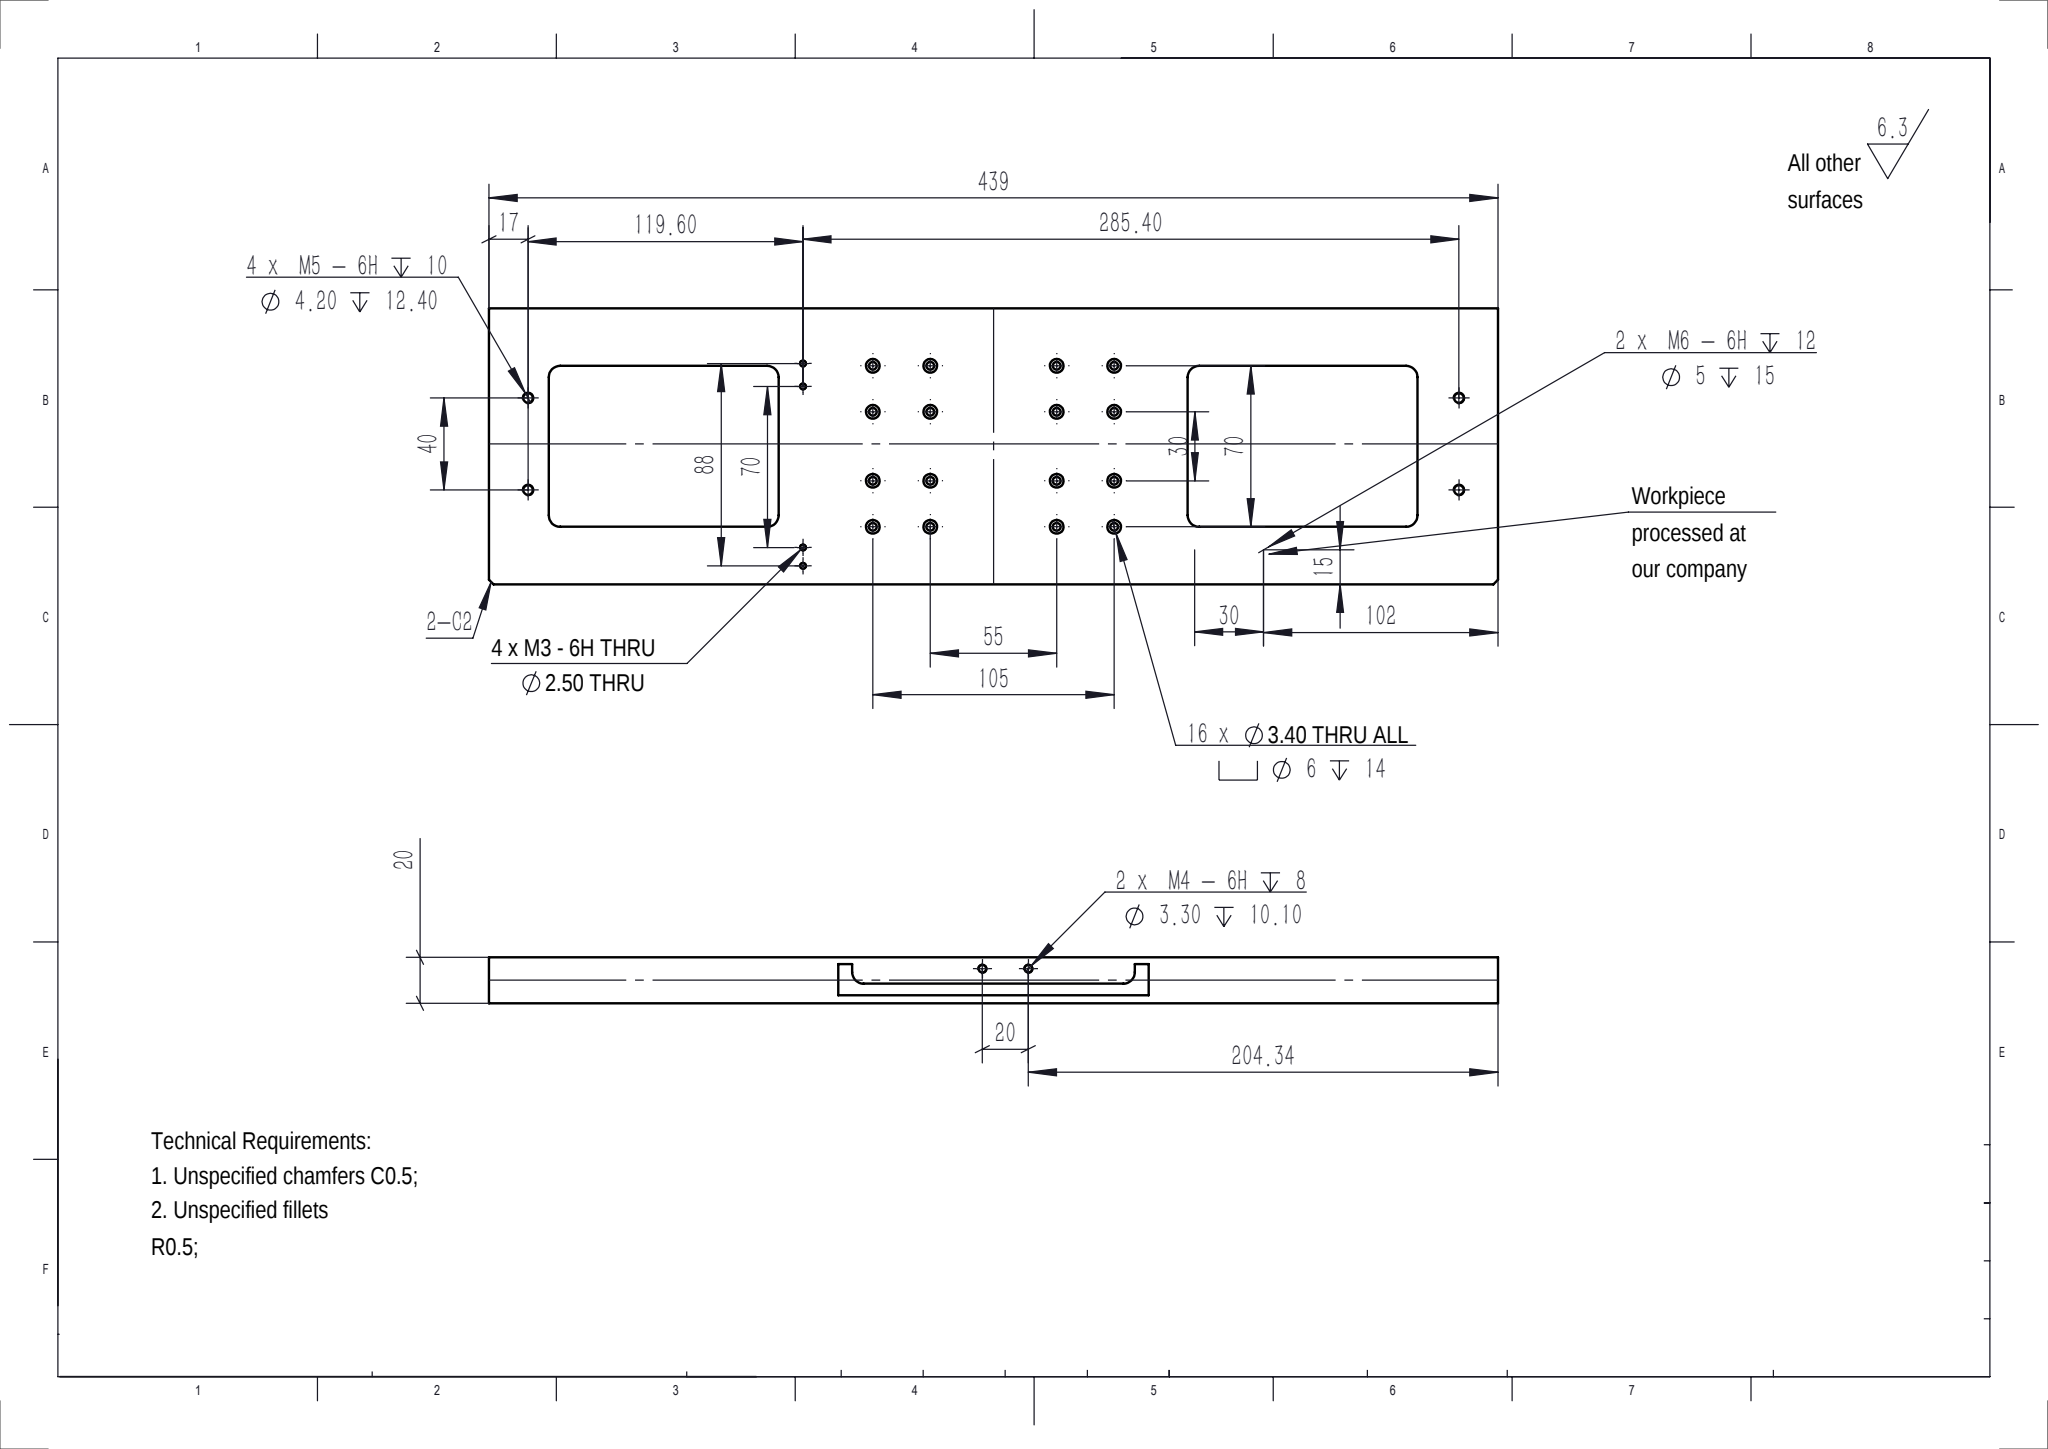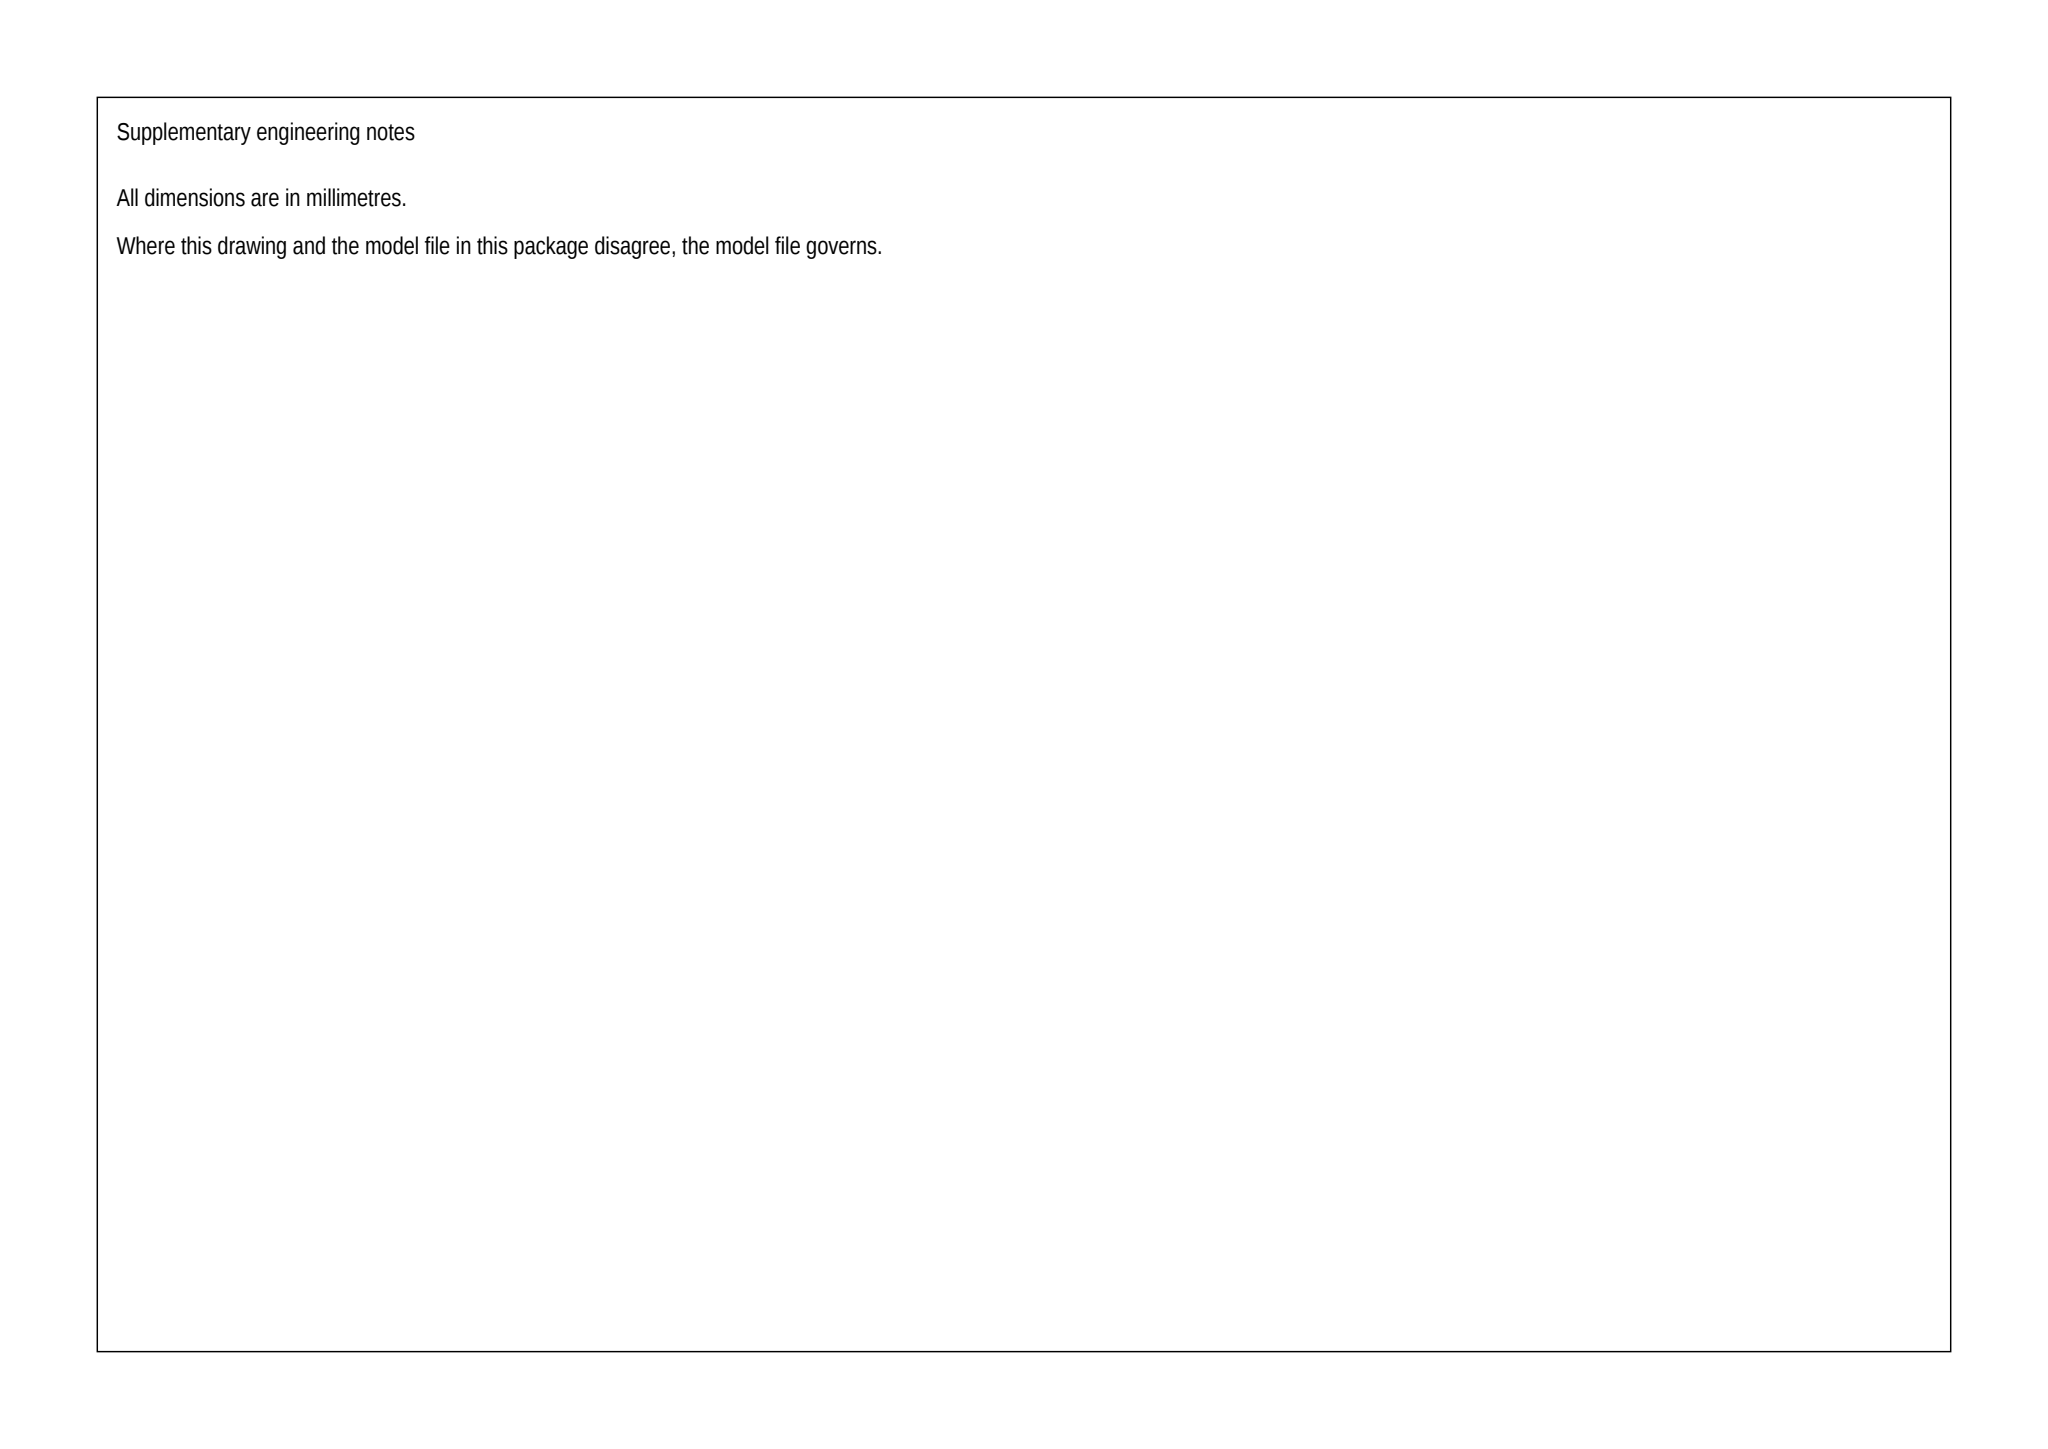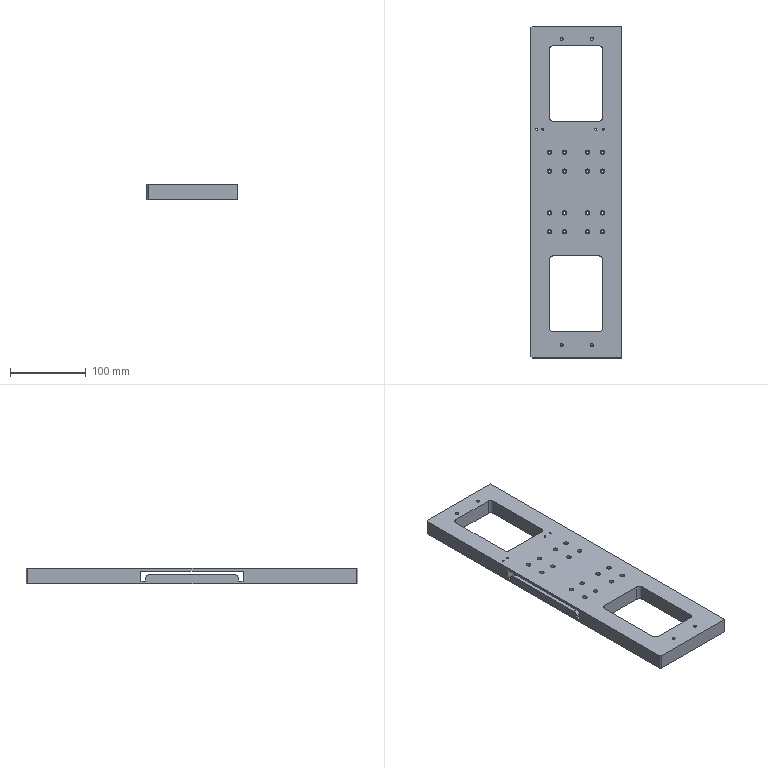Part | SolidWorks | mm | 1 solid | 186 faces | box 120 x 439 x 20 mm | volume 673017 mm3 | cylinder 130 | plane 40 | cone 16 | commonest cylinder face diameters 6 x64 3.4 x32 10 x10 2.5 x8 4.2 x8 5 x4 3.3 x4